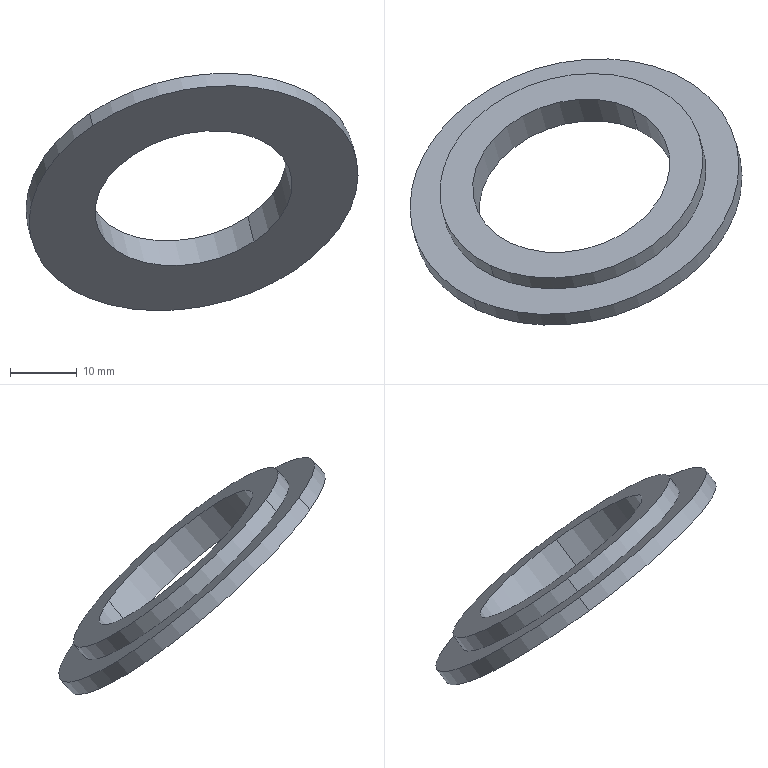Component | SolidWorks | FlatWasher15x50x2.5-7 | 1 solid | 9 faces | box 49.58 x 39.82 x 35.44 mm | volume 4516 mm3 | cylinder 6 | plane 3 | commonest cylinder face diameters 40 x2 30 x2 50 x2 | material Copper
build123d program:
from build123d import *

# Parameters (mm, degrees)
SKETCH1_R           = 25
SKETCH1_R_2         = 20
BOSS_EXTRUDE1_DEPTH = 2.5
SKETCH1_3_R         = 20
SKETCH1_3_R_2       = 15
BOSS_EXTRUDE2_DEPTH = 5


with BuildPart() as part:
    # Sketch1 → Boss-Extrude1 (new body)
    with BuildSketch(Plane(origin=(0, 0, 0), x_dir=(1, 0, 0), z_dir=(0, 1, 0))):
        with Locations(Location((0, 0, 0), (0, 0, 270))):
            Circle(SKETCH1_R)
        with Locations(Location((0, 0, 0), (0, 0, 270))):
            Circle(SKETCH1_R_2, mode=Mode.SUBTRACT)
    extrude(amount=BOSS_EXTRUDE1_DEPTH)

    # Sketch1_3 → Boss-Extrude2 (add)
    with BuildSketch(Plane(origin=(0, 0, 0), x_dir=(1, 0, 0), z_dir=(0, 1, 0))):
        with Locations(Location((0, 0, 0), (0, 0, 270))):
            Circle(SKETCH1_3_R)
        with Locations(Location((0, 0, 0), (0, 0, 270))):
            Circle(SKETCH1_3_R_2, mode=Mode.SUBTRACT)
    extrude(amount=BOSS_EXTRUDE2_DEPTH)


solid = part.part

# Placed as in the assembly
solid = solid.moved(Location((561.837, -2240.898, 662.657), (-145.668, -52.862, 161.876)))
STEP:
#1=CARTESIAN_POINT('',(22.557,-87.569,25.895));
#2=VERTEX_POINT('',#1);
#3=CARTESIAN_POINT('',(21.609,-88.626,26.575));
#4=VERTEX_POINT('',#3);
#5=CARTESIAN_POINT('',(22.083,-88.097,26.235));
#6=DIRECTION('',(-0.1878,0.645,0.7408));
#7=DIRECTION('',(0.602,0.6715,-0.432));
#8=AXIS2_PLACEMENT_3D('',#5,#6,#7);
#9=CIRCLE('',#8,0.7874);
#10=EDGE_CURVE('',#2,#4,#9,.T.);
#11=ORIENTED_EDGE('',*,*,#10,.F.);
#12=CARTESIAN_POINT('',(22.575,-87.632,25.822));
#13=VERTEX_POINT('',#12);
#14=CARTESIAN_POINT('',(22.557,-87.569,25.895));
#15=DIRECTION('',(0.1878,-0.645,-0.7408));
#16=VECTOR('',#15,39.37);
#17=LINE('',#14,#16);
#18=EDGE_CURVE('',#2,#13,#17,.T.);
#19=ORIENTED_EDGE('',*,*,#18,.T.);
#20=CARTESIAN_POINT('',(21.627,-88.69,26.502));
#21=VERTEX_POINT('',#20);
#22=CARTESIAN_POINT('',(22.101,-88.161,26.162));
#23=DIRECTION('',(-0.1878,0.645,0.7408));
#24=DIRECTION('',(0.602,0.6715,-0.432));
#25=AXIS2_PLACEMENT_3D('',#22,#23,#24);
#26=CIRCLE('',#25,0.7874);
#27=EDGE_CURVE('',#13,#21,#26,.T.);
#28=ORIENTED_EDGE('',*,*,#27,.T.);
#29=CARTESIAN_POINT('',(21.609,-88.626,26.575));
#30=DIRECTION('',(0.1878,-0.645,-0.7408));
#31=VECTOR('',#30,39.37);
#32=LINE('',#29,#31);
#33=EDGE_CURVE('',#4,#21,#32,.T.);
#34=ORIENTED_EDGE('',*,*,#33,.F.);
#35=EDGE_LOOP('',(#11,#19,#28,#34));
#36=FACE_OUTER_BOUND('',#35,.T.);
#37=CARTESIAN_POINT('',(22.083,-88.097,26.235));
#38=DIRECTION('',(0.1878,-0.645,-0.7408));
#39=DIRECTION('',(-0.602,-0.6715,0.432));
#40=AXIS2_PLACEMENT_3D('',#37,#38,#39);
#41=CYLINDRICAL_SURFACE('',#40,0.7874);
#42=ADVANCED_FACE('',(#36),#41,.T.);
#43=CARTESIAN_POINT('',(21.727,-88.494,26.49));
#44=VERTEX_POINT('',#43);
#45=CARTESIAN_POINT('',(22.438,-87.701,25.98));
#46=VERTEX_POINT('',#45);
#47=CARTESIAN_POINT('',(22.083,-88.097,26.235));
#48=DIRECTION('',(-0.1878,0.645,0.7408));
#49=DIRECTION('',(0.602,0.6715,-0.432));
#50=AXIS2_PLACEMENT_3D('',#47,#48,#49);
#51=CIRCLE('',#50,0.5906);
#52=EDGE_CURVE('',#44,#46,#51,.T.);
#53=ORIENTED_EDGE('',*,*,#52,.T.);
#54=CARTESIAN_POINT('',(22.475,-87.828,25.834));
#55=VERTEX_POINT('',#54);
#56=CARTESIAN_POINT('',(22.438,-87.701,25.98));
#57=DIRECTION('',(0.1878,-0.645,-0.7408));
#58=VECTOR('',#57,39.37);
#59=LINE('',#56,#58);
#60=EDGE_CURVE('',#46,#55,#59,.T.);
#61=ORIENTED_EDGE('',*,*,#60,.T.);
#62=CARTESIAN_POINT('',(21.764,-88.621,26.344));
#63=VERTEX_POINT('',#62);
#64=CARTESIAN_POINT('',(22.12,-88.224,26.089));
#65=DIRECTION('',(-0.1878,0.645,0.7408));
#66=DIRECTION('',(0.602,0.6715,-0.432));
#67=AXIS2_PLACEMENT_3D('',#64,#65,#66);
#68=CIRCLE('',#67,0.5906);
#69=EDGE_CURVE('',#63,#55,#68,.T.);
#70=ORIENTED_EDGE('',*,*,#69,.F.);
#71=CARTESIAN_POINT('',(21.727,-88.494,26.49));
#72=DIRECTION('',(0.1878,-0.645,-0.7408));
#73=VECTOR('',#72,39.37);
#74=LINE('',#71,#73);
#75=EDGE_CURVE('',#44,#63,#74,.T.);
#76=ORIENTED_EDGE('',*,*,#75,.F.);
#77=EDGE_LOOP('',(#53,#61,#70,#76));
#78=FACE_OUTER_BOUND('',#77,.T.);
#79=CARTESIAN_POINT('',(22.083,-88.097,26.235));
#80=DIRECTION('',(0.1878,-0.645,-0.7408));
#81=DIRECTION('',(-0.602,-0.6715,0.432));
#82=AXIS2_PLACEMENT_3D('',#79,#80,#81);
#83=CYLINDRICAL_SURFACE('',#82,0.5906);
#84=ADVANCED_FACE('',(#78),#83,.F.);
#85=CARTESIAN_POINT('',(22.694,-87.5,25.737));
#86=VERTEX_POINT('',#85);
#87=CARTESIAN_POINT('',(21.509,-88.822,26.587));
#88=VERTEX_POINT('',#87);
#89=CARTESIAN_POINT('',(22.101,-88.161,26.162));
#90=DIRECTION('',(-0.1878,0.645,0.7408));
#91=DIRECTION('',(0.602,0.6715,-0.432));
#92=AXIS2_PLACEMENT_3D('',#89,#90,#91);
#93=CIRCLE('',#92,0.9843);
#94=EDGE_CURVE('',#86,#88,#93,.T.);
#95=ORIENTED_EDGE('',*,*,#94,.F.);
#96=CARTESIAN_POINT('',(22.712,-87.563,25.664));
#97=VERTEX_POINT('',#96);
#98=CARTESIAN_POINT('',(22.694,-87.5,25.737));
#99=DIRECTION('',(0.1878,-0.645,-0.7408));
#100=VECTOR('',#99,39.37);
#101=LINE('',#98,#100);
#102=EDGE_CURVE('',#86,#97,#101,.T.);
#103=ORIENTED_EDGE('',*,*,#102,.T.);
#104=CARTESIAN_POINT('',(21.527,-88.885,26.514));
#105=VERTEX_POINT('',#104);
#106=CARTESIAN_POINT('',(22.12,-88.224,26.089));
#107=DIRECTION('',(-0.1878,0.645,0.7408));
#108=DIRECTION('',(0.602,0.6715,-0.432));
#109=AXIS2_PLACEMENT_3D('',#106,#107,#108);
#110=CIRCLE('',#109,0.9843);
#111=EDGE_CURVE('',#97,#105,#110,.T.);
#112=ORIENTED_EDGE('',*,*,#111,.T.);
#113=CARTESIAN_POINT('',(21.509,-88.822,26.587));
#114=DIRECTION('',(0.1878,-0.645,-0.7408));
#115=VECTOR('',#114,39.37);
#116=LINE('',#113,#115);
#117=EDGE_CURVE('',#88,#105,#116,.T.);
#118=ORIENTED_EDGE('',*,*,#117,.F.);
#119=EDGE_LOOP('',(#95,#103,#112,#118));
#120=FACE_OUTER_BOUND('',#119,.T.);
#121=CARTESIAN_POINT('',(22.101,-88.161,26.162));
#122=DIRECTION('',(0.1878,-0.645,-0.7408));
#123=DIRECTION('',(-0.602,-0.6715,0.432));
#124=AXIS2_PLACEMENT_3D('',#121,#122,#123);
#125=CYLINDRICAL_SURFACE('',#124,0.9843);
#126=ADVANCED_FACE('',(#120),#125,.T.);
#127=ORIENTED_EDGE('',*,*,#102,.F.);
#128=CARTESIAN_POINT('',(22.101,-88.161,26.162));
#129=DIRECTION('',(-0.1878,0.645,0.7408));
#130=DIRECTION('',(0.602,0.6715,-0.432));
#131=AXIS2_PLACEMENT_3D('',#128,#129,#130);
#132=CIRCLE('',#131,0.9843);
#133=EDGE_CURVE('',#88,#86,#132,.T.);
#134=ORIENTED_EDGE('',*,*,#133,.F.);
#135=ORIENTED_EDGE('',*,*,#117,.T.);
#136=CARTESIAN_POINT('',(22.12,-88.224,26.089));
#137=DIRECTION('',(-0.1878,0.645,0.7408));
#138=DIRECTION('',(0.602,0.6715,-0.432));
#139=AXIS2_PLACEMENT_3D('',#136,#137,#138);
#140=CIRCLE('',#139,0.9843);
#141=EDGE_CURVE('',#105,#97,#140,.T.);
#142=ORIENTED_EDGE('',*,*,#141,.T.);
#143=EDGE_LOOP('',(#127,#134,#135,#142));
#144=FACE_OUTER_BOUND('',#143,.T.);
#145=CARTESIAN_POINT('',(22.101,-88.161,26.162));
#146=DIRECTION('',(0.1878,-0.645,-0.7408));
#147=DIRECTION('',(-0.602,-0.6715,0.432));
#148=AXIS2_PLACEMENT_3D('',#145,#146,#147);
#149=CYLINDRICAL_SURFACE('',#148,0.9843);
#150=ADVANCED_FACE('',(#144),#149,.T.);
#151=CARTESIAN_POINT('',(22.101,-88.161,26.162));
#152=DIRECTION('',(-0.1878,0.645,0.7408));
#153=DIRECTION('',(0.602,0.6715,-0.432));
#154=AXIS2_PLACEMENT_3D('',#151,#152,#153);
#155=CIRCLE('',#154,0.7874);
#156=EDGE_CURVE('',#21,#13,#155,.T.);
#157=ORIENTED_EDGE('',*,*,#156,.F.);
#158=ORIENTED_EDGE('',*,*,#27,.F.);
#159=EDGE_LOOP('',(#157,#158));
#160=FACE_BOUND('',#159,.T.);
#161=ORIENTED_EDGE('',*,*,#133,.T.);
#162=ORIENTED_EDGE('',*,*,#94,.T.);
#163=EDGE_LOOP('',(#161,#162));
#164=FACE_OUTER_BOUND('',#163,.T.);
#165=CARTESIAN_POINT('',(22.101,-88.161,26.162));
#166=DIRECTION('',(-0.1878,0.645,0.7408));
#167=DIRECTION('',(0.602,0.6715,-0.432));
#168=AXIS2_PLACEMENT_3D('',#165,#166,#167);
#169=PLANE('',#168);
#170=ADVANCED_FACE('',(#160,#164),#169,.T.);
#171=ORIENTED_EDGE('',*,*,#141,.F.);
#172=ORIENTED_EDGE('',*,*,#111,.F.);
#173=EDGE_LOOP('',(#171,#172));
#174=FACE_OUTER_BOUND('',#173,.T.);
#175=ORIENTED_EDGE('',*,*,#69,.T.);
#176=CARTESIAN_POINT('',(22.12,-88.224,26.089));
#177=DIRECTION('',(-0.1878,0.645,0.7408));
#178=DIRECTION('',(0.602,0.6715,-0.432));
#179=AXIS2_PLACEMENT_3D('',#176,#177,#178);
#180=CIRCLE('',#179,0.5906);
#181=EDGE_CURVE('',#55,#63,#180,.T.);
#182=ORIENTED_EDGE('',*,*,#181,.T.);
#183=EDGE_LOOP('',(#175,#182));
#184=FACE_BOUND('',#183,.T.);
#185=CARTESIAN_POINT('',(22.12,-88.224,26.089));
#186=DIRECTION('',(-0.1878,0.645,0.7408));
#187=DIRECTION('',(0.602,0.6715,-0.432));
#188=AXIS2_PLACEMENT_3D('',#185,#186,#187);
#189=PLANE('',#188);
#190=ADVANCED_FACE('',(#174,#184),#189,.F.);
#191=ORIENTED_EDGE('',*,*,#60,.F.);
#192=CARTESIAN_POINT('',(22.083,-88.097,26.235));
#193=DIRECTION('',(-0.1878,0.645,0.7408));
#194=DIRECTION('',(0.602,0.6715,-0.432));
#195=AXIS2_PLACEMENT_3D('',#192,#193,#194);
#196=CIRCLE('',#195,0.5906);
#197=EDGE_CURVE('',#46,#44,#196,.T.);
#198=ORIENTED_EDGE('',*,*,#197,.T.);
#199=ORIENTED_EDGE('',*,*,#75,.T.);
#200=ORIENTED_EDGE('',*,*,#181,.F.);
#201=EDGE_LOOP('',(#191,#198,#199,#200));
#202=FACE_OUTER_BOUND('',#201,.T.);
#203=CARTESIAN_POINT('',(22.083,-88.097,26.235));
#204=DIRECTION('',(0.1878,-0.645,-0.7408));
#205=DIRECTION('',(-0.602,-0.6715,0.432));
#206=AXIS2_PLACEMENT_3D('',#203,#204,#205);
#207=CYLINDRICAL_SURFACE('',#206,0.5906);
#208=ADVANCED_FACE('',(#202),#207,.F.);
#209=ORIENTED_EDGE('',*,*,#18,.F.);
#210=CARTESIAN_POINT('',(22.083,-88.097,26.235));
#211=DIRECTION('',(-0.1878,0.645,0.7408));
#212=DIRECTION('',(0.602,0.6715,-0.432));
#213=AXIS2_PLACEMENT_3D('',#210,#211,#212);
#214=CIRCLE('',#213,0.7874);
#215=EDGE_CURVE('',#4,#2,#214,.T.);
#216=ORIENTED_EDGE('',*,*,#215,.F.);
#217=ORIENTED_EDGE('',*,*,#33,.T.);
#218=ORIENTED_EDGE('',*,*,#156,.T.);
#219=EDGE_LOOP('',(#209,#216,#217,#218));
#220=FACE_OUTER_BOUND('',#219,.T.);
#221=CARTESIAN_POINT('',(22.083,-88.097,26.235));
#222=DIRECTION('',(0.1878,-0.645,-0.7408));
#223=DIRECTION('',(-0.602,-0.6715,0.432));
#224=AXIS2_PLACEMENT_3D('',#221,#222,#223);
#225=CYLINDRICAL_SURFACE('',#224,0.7874);
#226=ADVANCED_FACE('',(#220),#225,.T.);
#227=ORIENTED_EDGE('',*,*,#52,.F.);
#228=ORIENTED_EDGE('',*,*,#197,.F.);
#229=EDGE_LOOP('',(#227,#228));
#230=FACE_BOUND('',#229,.T.);
#231=ORIENTED_EDGE('',*,*,#215,.T.);
#232=ORIENTED_EDGE('',*,*,#10,.T.);
#233=EDGE_LOOP('',(#231,#232));
#234=FACE_OUTER_BOUND('',#233,.T.);
#235=CARTESIAN_POINT('',(22.083,-88.097,26.235));
#236=DIRECTION('',(-0.1878,0.645,0.7408));
#237=DIRECTION('',(0.602,0.6715,-0.432));
#238=AXIS2_PLACEMENT_3D('',#235,#236,#237);
#239=PLANE('',#238);
#240=ADVANCED_FACE('',(#230,#234),#239,.T.);
#241=CLOSED_SHELL('',(#42,#84,#126,#150,#170,#190,#208,#226,#240));
#242=MANIFOLD_SOLID_BREP('',#241);
#243=CARTESIAN_POINT('',(0.,0.,0.));
#244=DIRECTION('',(0.,0.,1.));
#245=DIRECTION('',(1.,0.,0.));
#246=AXIS2_PLACEMENT_3D('',#243,#244,#245);
#247=(LENGTH_UNIT()NAMED_UNIT(*)SI_UNIT($,.METRE.));
#248=LENGTH_MEASURE_WITH_UNIT(LENGTH_MEASURE(0.0254),#247);
#249=DIMENSIONAL_EXPONENTS(1.,0.,0.,0.,0.,0.,0.);
#250=(CONVERSION_BASED_UNIT('',#248)LENGTH_UNIT()NAMED_UNIT(#249));
#251=UNCERTAINTY_MEASURE_WITH_UNIT(LENGTH_MEASURE(0.00001),#250,'','');
#252=(NAMED_UNIT(*)PLANE_ANGLE_UNIT()SI_UNIT($,.RADIAN.));
#253=(NAMED_UNIT(*)SI_UNIT($,.STERADIAN.)SOLID_ANGLE_UNIT());
#254=(GEOMETRIC_REPRESENTATION_CONTEXT(3)GLOBAL_UNCERTAINTY_ASSIGNED_CONTEXT((#251))GLOBAL_UNIT_ASSIGNED_CONTEXT((#250,#252,#253))REPRESENTATION_CONTEXT('',''));
#255=ADVANCED_BREP_SHAPE_REPRESENTATION('',(#242,#246),#254);
#256=COLOUR_RGB('',0.7922,0.8196,0.9333);
#257=FILL_AREA_STYLE_COLOUR('',#256);
#258=FILL_AREA_STYLE('',(#257));
#259=SURFACE_STYLE_FILL_AREA(#258);
#260=SURFACE_SIDE_STYLE('',(#259));
#261=SURFACE_STYLE_USAGE(.BOTH.,#260);
#262=PRESENTATION_STYLE_ASSIGNMENT((#261));
#263=STYLED_ITEM('',(#262),#242);
#264=PRESENTATION_LAYER_ASSIGNMENT('','',(#263));
#265=(LENGTH_UNIT()NAMED_UNIT(*)SI_UNIT($,.METRE.));
#266=LENGTH_MEASURE_WITH_UNIT(LENGTH_MEASURE(0.0254),#265);
#267=DIMENSIONAL_EXPONENTS(1.,0.,0.,0.,0.,0.,0.);
#268=(CONVERSION_BASED_UNIT('',#266)LENGTH_UNIT()NAMED_UNIT(#267));
#269=UNCERTAINTY_MEASURE_WITH_UNIT(LENGTH_MEASURE(0.00001),#268,'','');
#270=(NAMED_UNIT(*)PLANE_ANGLE_UNIT()SI_UNIT($,.RADIAN.));
#271=(NAMED_UNIT(*)SI_UNIT($,.STERADIAN.)SOLID_ANGLE_UNIT());
#272=(GEOMETRIC_REPRESENTATION_CONTEXT(3)GLOBAL_UNCERTAINTY_ASSIGNED_CONTEXT((#269))GLOBAL_UNIT_ASSIGNED_CONTEXT((#268,#270,#271))REPRESENTATION_CONTEXT('',''));
#273=MECHANICAL_DESIGN_GEOMETRIC_PRESENTATION_REPRESENTATION('',(#263),#272);